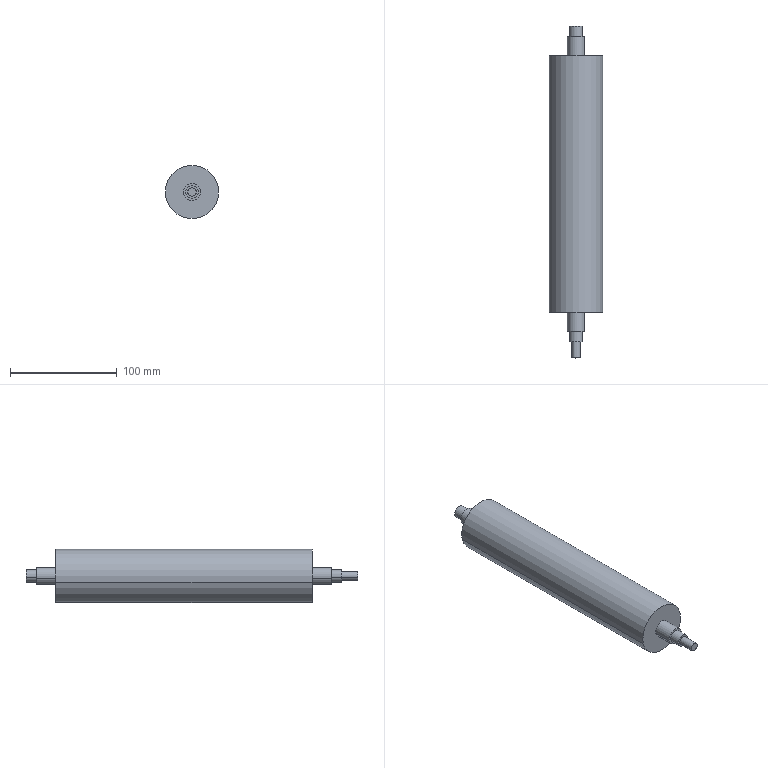Component | SolidWorks | AdjustmentRing-2 | 2 solids | 19 faces | box 50 x 311 x 50 mm | volume 481493 mm3 | cylinder 12 | plane 7 | commonest cylinder face diameters 16 x4 12 x4 50 x2 8 x2
build123d program:
from build123d import *

# Parameters (mm, degrees)
SKETCH4_R           = 25
SKETCH4_R_2         = 8
BOSS_EXTRUDE3_DEPTH = 120


with BuildPart() as part:
    # Sketch1 → Revolve1 (revolve)
    with BuildSketch(Plane.XY, mode=Mode.PRIVATE) as revolve1_sk:
        Polygon((0, 0), (6, 0), (6, 10), (8, 10), (8, 286), (6, 286), (6, 296), (4, 296), (4, 311), (0, 311), align=None)
    revolve(revolve1_sk.sketch.rotate(Axis((0, 0, 0), (0, 1, 0)), 90), axis=Axis((0, 0, 0), (0, 1, 0)))


with BuildPart() as body_2:
    # Sketch4 → Boss-Extrude3 (new, symmetric)
    with BuildSketch(Plane(origin=(0, 148, 0), x_dir=(-1, 0, 0), z_dir=(0, -1, 0))):
        with Locations(Location((0, 0, 0), (0, 0, 90))):
            Circle(SKETCH4_R)
        with Locations(Location((0, 0, 0), (0, 0, 90))):
            Circle(SKETCH4_R_2, mode=Mode.SUBTRACT)
    extrude(amount=BOSS_EXTRUDE3_DEPTH, both=True)


solid = Compound([part.part, body_2.part])

# Placed as in the assembly
solid = solid.moved(Location((-35, 148, 0), (180, 0, 0)))
STEP:
#1=COLOUR_RGB('',0.7922,0.8196,0.9333);
#2=FILL_AREA_STYLE_COLOUR('',#1);
#3=FILL_AREA_STYLE('',(#2));
#4=SURFACE_STYLE_FILL_AREA(#3);
#5=SURFACE_SIDE_STYLE('',(#4));
#6=SURFACE_STYLE_USAGE(.BOTH.,#5);
#7=PRESENTATION_STYLE_ASSIGNMENT((#6));
#8=CARTESIAN_POINT('',(-1.531,-6.417,-0.0381));
#9=VERTEX_POINT('',#8);
#10=CARTESIAN_POINT('',(-1.225,-6.417,0.0381));
#11=VERTEX_POINT('',#10);
#12=CARTESIAN_POINT('',(-1.378,-6.417,0.));
#13=DIRECTION('',(0.,1.,-0.));
#14=DIRECTION('',(-0.9703,0.,-0.2419));
#15=AXIS2_PLACEMENT_3D('',#12,#13,#14);
#16=CIRCLE('',#15,0.1575);
#17=EDGE_CURVE('',#9,#11,#16,.T.);
#18=ORIENTED_EDGE('',*,*,#17,.T.);
#19=CARTESIAN_POINT('',(-1.225,-5.827,0.0381));
#20=VERTEX_POINT('',#19);
#21=CARTESIAN_POINT('',(-1.225,5.827,0.0381));
#22=DIRECTION('',(0.,1.,-0.));
#23=VECTOR('',#22,39.37);
#24=LINE('',#21,#23);
#25=EDGE_CURVE('',#11,#20,#24,.T.);
#26=ORIENTED_EDGE('',*,*,#25,.T.);
#27=CARTESIAN_POINT('',(-1.531,-5.827,-0.0381));
#28=VERTEX_POINT('',#27);
#29=CARTESIAN_POINT('',(-1.378,-5.827,0.));
#30=DIRECTION('',(0.,1.,-0.));
#31=DIRECTION('',(-0.9703,0.,-0.2419));
#32=AXIS2_PLACEMENT_3D('',#29,#30,#31);
#33=CIRCLE('',#32,0.1575);
#34=EDGE_CURVE('',#28,#20,#33,.T.);
#35=ORIENTED_EDGE('',*,*,#34,.F.);
#36=CARTESIAN_POINT('',(-1.531,5.827,-0.0381));
#37=DIRECTION('',(0.,1.,-0.));
#38=VECTOR('',#37,39.37);
#39=LINE('',#36,#38);
#40=EDGE_CURVE('',#9,#28,#39,.T.);
#41=ORIENTED_EDGE('',*,*,#40,.F.);
#42=EDGE_LOOP('',(#18,#26,#35,#41));
#43=FACE_OUTER_BOUND('',#42,.T.);
#44=CARTESIAN_POINT('',(-1.378,5.827,0.));
#45=DIRECTION('',(0.,1.,-0.));
#46=DIRECTION('',(-0.9703,0.,-0.2419));
#47=AXIS2_PLACEMENT_3D('',#44,#45,#46);
#48=CYLINDRICAL_SURFACE('',#47,0.1575);
#49=ADVANCED_FACE('',(#43),#48,.T.);
#50=CARTESIAN_POINT('',(-1.607,-5.827,-0.05715));
#51=VERTEX_POINT('',#50);
#52=CARTESIAN_POINT('',(-1.149,-5.827,0.05715));
#53=VERTEX_POINT('',#52);
#54=CARTESIAN_POINT('',(-1.378,-5.827,0.));
#55=DIRECTION('',(0.,1.,-0.));
#56=DIRECTION('',(-0.9703,0.,-0.2419));
#57=AXIS2_PLACEMENT_3D('',#54,#55,#56);
#58=CIRCLE('',#57,0.2362);
#59=EDGE_CURVE('',#51,#53,#58,.T.);
#60=ORIENTED_EDGE('',*,*,#59,.T.);
#61=CARTESIAN_POINT('',(-1.149,-5.433,0.05715));
#62=VERTEX_POINT('',#61);
#63=CARTESIAN_POINT('',(-1.149,5.827,0.05715));
#64=DIRECTION('',(0.,1.,-0.));
#65=VECTOR('',#64,39.37);
#66=LINE('',#63,#65);
#67=EDGE_CURVE('',#53,#62,#66,.T.);
#68=ORIENTED_EDGE('',*,*,#67,.T.);
#69=CARTESIAN_POINT('',(-1.607,-5.433,-0.05715));
#70=VERTEX_POINT('',#69);
#71=CARTESIAN_POINT('',(-1.378,-5.433,0.));
#72=DIRECTION('',(0.,1.,-0.));
#73=DIRECTION('',(-0.9703,0.,-0.2419));
#74=AXIS2_PLACEMENT_3D('',#71,#72,#73);
#75=CIRCLE('',#74,0.2362);
#76=EDGE_CURVE('',#70,#62,#75,.T.);
#77=ORIENTED_EDGE('',*,*,#76,.F.);
#78=CARTESIAN_POINT('',(-1.607,5.827,-0.05715));
#79=DIRECTION('',(0.,1.,-0.));
#80=VECTOR('',#79,39.37);
#81=LINE('',#78,#80);
#82=EDGE_CURVE('',#51,#70,#81,.T.);
#83=ORIENTED_EDGE('',*,*,#82,.F.);
#84=EDGE_LOOP('',(#60,#68,#77,#83));
#85=FACE_OUTER_BOUND('',#84,.T.);
#86=CARTESIAN_POINT('',(-1.378,5.827,0.));
#87=DIRECTION('',(0.,1.,-0.));
#88=DIRECTION('',(-0.9703,0.,-0.2419));
#89=AXIS2_PLACEMENT_3D('',#86,#87,#88);
#90=CYLINDRICAL_SURFACE('',#89,0.2362);
#91=ADVANCED_FACE('',(#85),#90,.T.);
#92=CARTESIAN_POINT('',(-1.684,-5.433,-0.0762));
#93=VERTEX_POINT('',#92);
#94=CARTESIAN_POINT('',(-1.072,-5.433,0.0762));
#95=VERTEX_POINT('',#94);
#96=CARTESIAN_POINT('',(-1.378,-5.433,0.));
#97=DIRECTION('',(0.,1.,-0.));
#98=DIRECTION('',(-0.9703,0.,-0.2419));
#99=AXIS2_PLACEMENT_3D('',#96,#97,#98);
#100=CIRCLE('',#99,0.315);
#101=EDGE_CURVE('',#93,#95,#100,.T.);
#102=ORIENTED_EDGE('',*,*,#101,.T.);
#103=CARTESIAN_POINT('',(-1.072,5.433,0.0762));
#104=VERTEX_POINT('',#103);
#105=CARTESIAN_POINT('',(-1.072,5.827,0.0762));
#106=DIRECTION('',(0.,1.,-0.));
#107=VECTOR('',#106,39.37);
#108=LINE('',#105,#107);
#109=EDGE_CURVE('',#95,#104,#108,.T.);
#110=ORIENTED_EDGE('',*,*,#109,.T.);
#111=CARTESIAN_POINT('',(-1.684,5.433,-0.0762));
#112=VERTEX_POINT('',#111);
#113=CARTESIAN_POINT('',(-1.378,5.433,0.));
#114=DIRECTION('',(0.,1.,-0.));
#115=DIRECTION('',(-0.9703,0.,-0.2419));
#116=AXIS2_PLACEMENT_3D('',#113,#114,#115);
#117=CIRCLE('',#116,0.315);
#118=EDGE_CURVE('',#112,#104,#117,.T.);
#119=ORIENTED_EDGE('',*,*,#118,.F.);
#120=CARTESIAN_POINT('',(-1.684,5.827,-0.0762));
#121=DIRECTION('',(0.,1.,-0.));
#122=VECTOR('',#121,39.37);
#123=LINE('',#120,#122);
#124=EDGE_CURVE('',#93,#112,#123,.T.);
#125=ORIENTED_EDGE('',*,*,#124,.F.);
#126=EDGE_LOOP('',(#102,#110,#119,#125));
#127=FACE_OUTER_BOUND('',#126,.T.);
#128=CARTESIAN_POINT('',(-1.378,5.827,0.));
#129=DIRECTION('',(0.,1.,-0.));
#130=DIRECTION('',(-0.9703,0.,-0.2419));
#131=AXIS2_PLACEMENT_3D('',#128,#129,#130);
#132=CYLINDRICAL_SURFACE('',#131,0.315);
#133=ADVANCED_FACE('',(#127),#132,.T.);
#134=CARTESIAN_POINT('',(-1.607,5.433,-0.05715));
#135=VERTEX_POINT('',#134);
#136=CARTESIAN_POINT('',(-1.149,5.433,0.05715));
#137=VERTEX_POINT('',#136);
#138=CARTESIAN_POINT('',(-1.378,5.433,0.));
#139=DIRECTION('',(0.,1.,-0.));
#140=DIRECTION('',(-0.9703,0.,-0.2419));
#141=AXIS2_PLACEMENT_3D('',#138,#139,#140);
#142=CIRCLE('',#141,0.2362);
#143=EDGE_CURVE('',#135,#137,#142,.T.);
#144=ORIENTED_EDGE('',*,*,#143,.T.);
#145=CARTESIAN_POINT('',(-1.149,5.827,0.05715));
#146=VERTEX_POINT('',#145);
#147=CARTESIAN_POINT('',(-1.149,5.827,0.05715));
#148=DIRECTION('',(0.,1.,-0.));
#149=VECTOR('',#148,39.37);
#150=LINE('',#147,#149);
#151=EDGE_CURVE('',#137,#146,#150,.T.);
#152=ORIENTED_EDGE('',*,*,#151,.T.);
#153=CARTESIAN_POINT('',(-1.607,5.827,-0.05715));
#154=VERTEX_POINT('',#153);
#155=CARTESIAN_POINT('',(-1.378,5.827,0.));
#156=DIRECTION('',(0.,1.,-0.));
#157=DIRECTION('',(-0.9703,0.,-0.2419));
#158=AXIS2_PLACEMENT_3D('',#155,#156,#157);
#159=CIRCLE('',#158,0.2362);
#160=EDGE_CURVE('',#154,#146,#159,.T.);
#161=ORIENTED_EDGE('',*,*,#160,.F.);
#162=CARTESIAN_POINT('',(-1.607,5.827,-0.05715));
#163=DIRECTION('',(0.,1.,-0.));
#164=VECTOR('',#163,39.37);
#165=LINE('',#162,#164);
#166=EDGE_CURVE('',#135,#154,#165,.T.);
#167=ORIENTED_EDGE('',*,*,#166,.F.);
#168=EDGE_LOOP('',(#144,#152,#161,#167));
#169=FACE_OUTER_BOUND('',#168,.T.);
#170=CARTESIAN_POINT('',(-1.378,5.827,0.));
#171=DIRECTION('',(0.,1.,-0.));
#172=DIRECTION('',(-0.9703,0.,-0.2419));
#173=AXIS2_PLACEMENT_3D('',#170,#171,#172);
#174=CYLINDRICAL_SURFACE('',#173,0.2362);
#175=ADVANCED_FACE('',(#169),#174,.T.);
#176=ORIENTED_EDGE('',*,*,#160,.T.);
#177=CARTESIAN_POINT('',(-1.378,5.827,0.));
#178=DIRECTION('',(0.,1.,-0.));
#179=DIRECTION('',(-0.9703,0.,-0.2419));
#180=AXIS2_PLACEMENT_3D('',#177,#178,#179);
#181=CIRCLE('',#180,0.2362);
#182=EDGE_CURVE('',#146,#154,#181,.T.);
#183=ORIENTED_EDGE('',*,*,#182,.T.);
#184=EDGE_LOOP('',(#176,#183));
#185=FACE_OUTER_BOUND('',#184,.T.);
#186=CARTESIAN_POINT('',(-1.378,5.827,0.));
#187=DIRECTION('',(0.,1.,-0.));
#188=DIRECTION('',(-0.9703,-0.,-0.2419));
#189=AXIS2_PLACEMENT_3D('',#186,#187,#188);
#190=PLANE('',#189);
#191=ADVANCED_FACE('',(#185),#190,.T.);
#192=ORIENTED_EDGE('',*,*,#151,.F.);
#193=CARTESIAN_POINT('',(-1.378,5.433,0.));
#194=DIRECTION('',(0.,1.,-0.));
#195=DIRECTION('',(-0.9703,0.,-0.2419));
#196=AXIS2_PLACEMENT_3D('',#193,#194,#195);
#197=CIRCLE('',#196,0.2362);
#198=EDGE_CURVE('',#137,#135,#197,.T.);
#199=ORIENTED_EDGE('',*,*,#198,.T.);
#200=ORIENTED_EDGE('',*,*,#166,.T.);
#201=ORIENTED_EDGE('',*,*,#182,.F.);
#202=EDGE_LOOP('',(#192,#199,#200,#201));
#203=FACE_OUTER_BOUND('',#202,.T.);
#204=CARTESIAN_POINT('',(-1.378,5.827,0.));
#205=DIRECTION('',(0.,1.,-0.));
#206=DIRECTION('',(-0.9703,0.,-0.2419));
#207=AXIS2_PLACEMENT_3D('',#204,#205,#206);
#208=CYLINDRICAL_SURFACE('',#207,0.2362);
#209=ADVANCED_FACE('',(#203),#208,.T.);
#210=ORIENTED_EDGE('',*,*,#118,.T.);
#211=CARTESIAN_POINT('',(-1.378,5.433,0.));
#212=DIRECTION('',(0.,1.,-0.));
#213=DIRECTION('',(-0.9703,0.,-0.2419));
#214=AXIS2_PLACEMENT_3D('',#211,#212,#213);
#215=CIRCLE('',#214,0.315);
#216=EDGE_CURVE('',#104,#112,#215,.T.);
#217=ORIENTED_EDGE('',*,*,#216,.T.);
#218=EDGE_LOOP('',(#210,#217));
#219=FACE_OUTER_BOUND('',#218,.T.);
#220=ORIENTED_EDGE('',*,*,#143,.F.);
#221=ORIENTED_EDGE('',*,*,#198,.F.);
#222=EDGE_LOOP('',(#220,#221));
#223=FACE_BOUND('',#222,.T.);
#224=CARTESIAN_POINT('',(-1.435,5.433,0.2292));
#225=DIRECTION('',(0.,1.,-0.));
#226=DIRECTION('',(-0.9703,-0.,-0.2419));
#227=AXIS2_PLACEMENT_3D('',#224,#225,#226);
#228=PLANE('',#227);
#229=ADVANCED_FACE('',(#219,#223),#228,.T.);
#230=ORIENTED_EDGE('',*,*,#109,.F.);
#231=CARTESIAN_POINT('',(-1.378,-5.433,0.));
#232=DIRECTION('',(0.,1.,-0.));
#233=DIRECTION('',(-0.9703,0.,-0.2419));
#234=AXIS2_PLACEMENT_3D('',#231,#232,#233);
#235=CIRCLE('',#234,0.315);
#236=EDGE_CURVE('',#95,#93,#235,.T.);
#237=ORIENTED_EDGE('',*,*,#236,.T.);
#238=ORIENTED_EDGE('',*,*,#124,.T.);
#239=ORIENTED_EDGE('',*,*,#216,.F.);
#240=EDGE_LOOP('',(#230,#237,#238,#239));
#241=FACE_OUTER_BOUND('',#240,.T.);
#242=CARTESIAN_POINT('',(-1.378,5.827,0.));
#243=DIRECTION('',(0.,1.,-0.));
#244=DIRECTION('',(-0.9703,0.,-0.2419));
#245=AXIS2_PLACEMENT_3D('',#242,#243,#244);
#246=CYLINDRICAL_SURFACE('',#245,0.315);
#247=ADVANCED_FACE('',(#241),#246,.T.);
#248=ORIENTED_EDGE('',*,*,#76,.T.);
#249=CARTESIAN_POINT('',(-1.378,-5.433,0.));
#250=DIRECTION('',(0.,1.,-0.));
#251=DIRECTION('',(-0.9703,0.,-0.2419));
#252=AXIS2_PLACEMENT_3D('',#249,#250,#251);
#253=CIRCLE('',#252,0.2362);
#254=EDGE_CURVE('',#62,#70,#253,.T.);
#255=ORIENTED_EDGE('',*,*,#254,.T.);
#256=EDGE_LOOP('',(#248,#255));
#257=FACE_BOUND('',#256,.T.);
#258=ORIENTED_EDGE('',*,*,#101,.F.);
#259=ORIENTED_EDGE('',*,*,#236,.F.);
#260=EDGE_LOOP('',(#258,#259));
#261=FACE_OUTER_BOUND('',#260,.T.);
#262=CARTESIAN_POINT('',(-1.454,-5.433,0.3056));
#263=DIRECTION('',(-0.,-1.,0.));
#264=DIRECTION('',(0.9703,0.,0.2419));
#265=AXIS2_PLACEMENT_3D('',#262,#263,#264);
#266=PLANE('',#265);
#267=ADVANCED_FACE('',(#257,#261),#266,.T.);
#268=ORIENTED_EDGE('',*,*,#67,.F.);
#269=CARTESIAN_POINT('',(-1.378,-5.827,0.));
#270=DIRECTION('',(0.,1.,-0.));
#271=DIRECTION('',(-0.9703,0.,-0.2419));
#272=AXIS2_PLACEMENT_3D('',#269,#270,#271);
#273=CIRCLE('',#272,0.2362);
#274=EDGE_CURVE('',#53,#51,#273,.T.);
#275=ORIENTED_EDGE('',*,*,#274,.T.);
#276=ORIENTED_EDGE('',*,*,#82,.T.);
#277=ORIENTED_EDGE('',*,*,#254,.F.);
#278=EDGE_LOOP('',(#268,#275,#276,#277));
#279=FACE_OUTER_BOUND('',#278,.T.);
#280=CARTESIAN_POINT('',(-1.378,5.827,0.));
#281=DIRECTION('',(0.,1.,-0.));
#282=DIRECTION('',(-0.9703,0.,-0.2419));
#283=AXIS2_PLACEMENT_3D('',#280,#281,#282);
#284=CYLINDRICAL_SURFACE('',#283,0.2362);
#285=ADVANCED_FACE('',(#279),#284,.T.);
#286=ORIENTED_EDGE('',*,*,#34,.T.);
#287=CARTESIAN_POINT('',(-1.378,-5.827,0.));
#288=DIRECTION('',(0.,1.,-0.));
#289=DIRECTION('',(-0.9703,0.,-0.2419));
#290=AXIS2_PLACEMENT_3D('',#287,#288,#289);
#291=CIRCLE('',#290,0.1575);
#292=EDGE_CURVE('',#20,#28,#291,.T.);
#293=ORIENTED_EDGE('',*,*,#292,.T.);
#294=EDGE_LOOP('',(#286,#293));
#295=FACE_BOUND('',#294,.T.);
#296=ORIENTED_EDGE('',*,*,#59,.F.);
#297=ORIENTED_EDGE('',*,*,#274,.F.);
#298=EDGE_LOOP('',(#296,#297));
#299=FACE_OUTER_BOUND('',#298,.T.);
#300=CARTESIAN_POINT('',(-1.435,-5.827,0.2292));
#301=DIRECTION('',(-0.,-1.,0.));
#302=DIRECTION('',(0.9703,0.,0.2419));
#303=AXIS2_PLACEMENT_3D('',#300,#301,#302);
#304=PLANE('',#303);
#305=ADVANCED_FACE('',(#295,#299),#304,.T.);
#306=ORIENTED_EDGE('',*,*,#25,.F.);
#307=CARTESIAN_POINT('',(-1.378,-6.417,0.));
#308=DIRECTION('',(0.,1.,-0.));
#309=DIRECTION('',(-0.9703,0.,-0.2419));
#310=AXIS2_PLACEMENT_3D('',#307,#308,#309);
#311=CIRCLE('',#310,0.1575);
#312=EDGE_CURVE('',#11,#9,#311,.T.);
#313=ORIENTED_EDGE('',*,*,#312,.T.);
#314=ORIENTED_EDGE('',*,*,#40,.T.);
#315=ORIENTED_EDGE('',*,*,#292,.F.);
#316=EDGE_LOOP('',(#306,#313,#314,#315));
#317=FACE_OUTER_BOUND('',#316,.T.);
#318=CARTESIAN_POINT('',(-1.378,5.827,0.));
#319=DIRECTION('',(0.,1.,-0.));
#320=DIRECTION('',(-0.9703,0.,-0.2419));
#321=AXIS2_PLACEMENT_3D('',#318,#319,#320);
#322=CYLINDRICAL_SURFACE('',#321,0.1575);
#323=ADVANCED_FACE('',(#317),#322,.T.);
#324=ORIENTED_EDGE('',*,*,#17,.F.);
#325=ORIENTED_EDGE('',*,*,#312,.F.);
#326=EDGE_LOOP('',(#324,#325));
#327=FACE_OUTER_BOUND('',#326,.T.);
#328=CARTESIAN_POINT('',(-1.416,-6.417,0.1528));
#329=DIRECTION('',(-0.,-1.,0.));
#330=DIRECTION('',(0.9703,0.,0.2419));
#331=AXIS2_PLACEMENT_3D('',#328,#329,#330);
#332=PLANE('',#331);
#333=ADVANCED_FACE('',(#327),#332,.T.);
#334=CLOSED_SHELL('',(#49,#91,#133,#175,#191,#209,#229,#247,#267,#285,#305,#323,#333));
#335=MANIFOLD_SOLID_BREP('',#334);
#336=STYLED_ITEM('',(#7),#335);
#337=PRESENTATION_LAYER_ASSIGNMENT('','',(#336));
#338=CARTESIAN_POINT('',(-1.072,4.724,0.0762));
#339=VERTEX_POINT('',#338);
#340=CARTESIAN_POINT('',(-1.684,4.724,-0.0762));
#341=VERTEX_POINT('',#340);
#342=CARTESIAN_POINT('',(-1.378,4.724,0.));
#343=DIRECTION('',(0.,1.,-0.));
#344=DIRECTION('',(-0.9703,0.,-0.2419));
#345=AXIS2_PLACEMENT_3D('',#342,#343,#344);
#346=CIRCLE('',#345,0.315);
#347=EDGE_CURVE('',#339,#341,#346,.T.);
#348=ORIENTED_EDGE('',*,*,#347,.T.);
#349=CARTESIAN_POINT('',(-1.684,-4.724,-0.0762));
#350=VERTEX_POINT('',#349);
#351=CARTESIAN_POINT('',(-1.684,4.724,-0.0762));
#352=DIRECTION('',(-0.,-1.,0.));
#353=VECTOR('',#352,39.37);
#354=LINE('',#351,#353);
#355=EDGE_CURVE('',#341,#350,#354,.T.);
#356=ORIENTED_EDGE('',*,*,#355,.T.);
#357=CARTESIAN_POINT('',(-1.072,-4.724,0.0762));
#358=VERTEX_POINT('',#357);
#359=CARTESIAN_POINT('',(-1.378,-4.724,0.));
#360=DIRECTION('',(0.,1.,-0.));
#361=DIRECTION('',(-0.9703,0.,-0.2419));
#362=AXIS2_PLACEMENT_3D('',#359,#360,#361);
#363=CIRCLE('',#362,0.315);
#364=EDGE_CURVE('',#358,#350,#363,.T.);
#365=ORIENTED_EDGE('',*,*,#364,.F.);
#366=CARTESIAN_POINT('',(-1.072,4.724,0.0762));
#367=DIRECTION('',(-0.,-1.,0.));
#368=VECTOR('',#367,39.37);
#369=LINE('',#366,#368);
#370=EDGE_CURVE('',#339,#358,#369,.T.);
#371=ORIENTED_EDGE('',*,*,#370,.F.);
#372=EDGE_LOOP('',(#348,#356,#365,#371));
#373=FACE_OUTER_BOUND('',#372,.T.);
#374=CARTESIAN_POINT('',(-1.378,4.724,0.));
#375=DIRECTION('',(-0.,-1.,0.));
#376=DIRECTION('',(0.9703,0.,0.2419));
#377=AXIS2_PLACEMENT_3D('',#374,#375,#376);
#378=CYLINDRICAL_SURFACE('',#377,0.315);
#379=ADVANCED_FACE('',(#373),#378,.F.);
#380=CARTESIAN_POINT('',(-2.333,4.724,-0.2381));
#381=VERTEX_POINT('',#380);
#382=CARTESIAN_POINT('',(-0.4229,4.724,0.2381));
#383=VERTEX_POINT('',#382);
#384=CARTESIAN_POINT('',(-1.378,4.724,0.));
#385=DIRECTION('',(0.,1.,-0.));
#386=DIRECTION('',(-0.9703,0.,-0.2419));
#387=AXIS2_PLACEMENT_3D('',#384,#385,#386);
#388=CIRCLE('',#387,0.9843);
#389=EDGE_CURVE('',#381,#383,#388,.T.);
#390=ORIENTED_EDGE('',*,*,#389,.F.);
#391=CARTESIAN_POINT('',(-2.333,-4.724,-0.2381));
#392=VERTEX_POINT('',#391);
#393=CARTESIAN_POINT('',(-2.333,4.724,-0.2381));
#394=DIRECTION('',(-0.,-1.,0.));
#395=VECTOR('',#394,39.37);
#396=LINE('',#393,#395);
#397=EDGE_CURVE('',#381,#392,#396,.T.);
#398=ORIENTED_EDGE('',*,*,#397,.T.);
#399=CARTESIAN_POINT('',(-0.4229,-4.724,0.2381));
#400=VERTEX_POINT('',#399);
#401=CARTESIAN_POINT('',(-1.378,-4.724,0.));
#402=DIRECTION('',(0.,1.,-0.));
#403=DIRECTION('',(-0.9703,0.,-0.2419));
#404=AXIS2_PLACEMENT_3D('',#401,#402,#403);
#405=CIRCLE('',#404,0.9843);
#406=EDGE_CURVE('',#392,#400,#405,.T.);
#407=ORIENTED_EDGE('',*,*,#406,.T.);
#408=CARTESIAN_POINT('',(-0.4229,4.724,0.2381));
#409=DIRECTION('',(-0.,-1.,0.));
#410=VECTOR('',#409,39.37);
#411=LINE('',#408,#410);
#412=EDGE_CURVE('',#383,#400,#411,.T.);
#413=ORIENTED_EDGE('',*,*,#412,.F.);
#414=EDGE_LOOP('',(#390,#398,#407,#413));
#415=FACE_OUTER_BOUND('',#414,.T.);
#416=CARTESIAN_POINT('',(-1.378,4.724,0.));
#417=DIRECTION('',(-0.,-1.,0.));
#418=DIRECTION('',(0.9703,0.,0.2419));
#419=AXIS2_PLACEMENT_3D('',#416,#417,#418);
#420=CYLINDRICAL_SURFACE('',#419,0.9843);
#421=ADVANCED_FACE('',(#415),#420,.T.);
#422=CARTESIAN_POINT('',(-1.378,4.724,0.));
#423=DIRECTION('',(0.,1.,-0.));
#424=DIRECTION('',(-0.9703,0.,-0.2419));
#425=AXIS2_PLACEMENT_3D('',#422,#423,#424);
#426=CIRCLE('',#425,0.9843);
#427=EDGE_CURVE('',#383,#381,#426,.T.);
#428=ORIENTED_EDGE('',*,*,#427,.T.);
#429=ORIENTED_EDGE('',*,*,#389,.T.);
#430=EDGE_LOOP('',(#428,#429));
#431=FACE_OUTER_BOUND('',#430,.T.);
#432=ORIENTED_EDGE('',*,*,#347,.F.);
#433=CARTESIAN_POINT('',(-1.378,4.724,0.));
#434=DIRECTION('',(0.,1.,-0.));
#435=DIRECTION('',(-0.9703,0.,-0.2419));
#436=AXIS2_PLACEMENT_3D('',#433,#434,#435);
#437=CIRCLE('',#436,0.315);
#438=EDGE_CURVE('',#341,#339,#437,.T.);
#439=ORIENTED_EDGE('',*,*,#438,.F.);
#440=EDGE_LOOP('',(#432,#439));
#441=FACE_BOUND('',#440,.T.);
#442=CARTESIAN_POINT('',(-1.378,4.724,0.));
#443=DIRECTION('',(0.,1.,-0.));
#444=DIRECTION('',(-0.9703,-0.,-0.2419));
#445=AXIS2_PLACEMENT_3D('',#442,#443,#444);
#446=PLANE('',#445);
#447=ADVANCED_FACE('',(#431,#441),#446,.T.);
#448=CARTESIAN_POINT('',(-1.378,-4.724,0.));
#449=DIRECTION('',(0.,1.,-0.));
#450=DIRECTION('',(-0.9703,0.,-0.2419));
#451=AXIS2_PLACEMENT_3D('',#448,#449,#450);
#452=CIRCLE('',#451,0.9843);
#453=EDGE_CURVE('',#400,#392,#452,.T.);
#454=ORIENTED_EDGE('',*,*,#453,.F.);
#455=ORIENTED_EDGE('',*,*,#406,.F.);
#456=EDGE_LOOP('',(#454,#455));
#457=FACE_OUTER_BOUND('',#456,.T.);
#458=ORIENTED_EDGE('',*,*,#364,.T.);
#459=CARTESIAN_POINT('',(-1.378,-4.724,0.));
#460=DIRECTION('',(0.,1.,-0.));
#461=DIRECTION('',(-0.9703,0.,-0.2419));
#462=AXIS2_PLACEMENT_3D('',#459,#460,#461);
#463=CIRCLE('',#462,0.315);
#464=EDGE_CURVE('',#350,#358,#463,.T.);
#465=ORIENTED_EDGE('',*,*,#464,.T.);
#466=EDGE_LOOP('',(#458,#465));
#467=FACE_BOUND('',#466,.T.);
#468=CARTESIAN_POINT('',(-1.378,-4.724,0.));
#469=DIRECTION('',(0.,1.,-0.));
#470=DIRECTION('',(-0.9703,-0.,-0.2419));
#471=AXIS2_PLACEMENT_3D('',#468,#469,#470);
#472=PLANE('',#471);
#473=ADVANCED_FACE('',(#457,#467),#472,.F.);
#474=ORIENTED_EDGE('',*,*,#397,.F.);
#475=ORIENTED_EDGE('',*,*,#427,.F.);
#476=ORIENTED_EDGE('',*,*,#412,.T.);
#477=ORIENTED_EDGE('',*,*,#453,.T.);
#478=EDGE_LOOP('',(#474,#475,#476,#477));
#479=FACE_OUTER_BOUND('',#478,.T.);
#480=CARTESIAN_POINT('',(-1.378,4.724,0.));
#481=DIRECTION('',(-0.,-1.,0.));
#482=DIRECTION('',(0.9703,0.,0.2419));
#483=AXIS2_PLACEMENT_3D('',#480,#481,#482);
#484=CYLINDRICAL_SURFACE('',#483,0.9843);
#485=ADVANCED_FACE('',(#479),#484,.T.);
#486=ORIENTED_EDGE('',*,*,#355,.F.);
#487=ORIENTED_EDGE('',*,*,#438,.T.);
#488=ORIENTED_EDGE('',*,*,#370,.T.);
#489=ORIENTED_EDGE('',*,*,#464,.F.);
#490=EDGE_LOOP('',(#486,#487,#488,#489));
#491=FACE_OUTER_BOUND('',#490,.T.);
#492=CARTESIAN_POINT('',(-1.378,4.724,0.));
#493=DIRECTION('',(-0.,-1.,0.));
#494=DIRECTION('',(0.9703,0.,0.2419));
#495=AXIS2_PLACEMENT_3D('',#492,#493,#494);
#496=CYLINDRICAL_SURFACE('',#495,0.315);
#497=ADVANCED_FACE('',(#491),#496,.F.);
#498=CLOSED_SHELL('',(#379,#421,#447,#473,#485,#497));
#499=MANIFOLD_SOLID_BREP('',#498);
#500=CARTESIAN_POINT('',(0.,0.,0.));
#501=DIRECTION('',(0.,0.,1.));
#502=DIRECTION('',(1.,0.,0.));
#503=AXIS2_PLACEMENT_3D('',#500,#501,#502);
#504=(LENGTH_UNIT()NAMED_UNIT(*)SI_UNIT($,.METRE.));
#505=LENGTH_MEASURE_WITH_UNIT(LENGTH_MEASURE(0.0254),#504);
#506=DIMENSIONAL_EXPONENTS(1.,0.,0.,0.,0.,0.,0.);
#507=(CONVERSION_BASED_UNIT('',#505)LENGTH_UNIT()NAMED_UNIT(#506));
#508=UNCERTAINTY_MEASURE_WITH_UNIT(LENGTH_MEASURE(0.00001),#507,'','');
#509=(NAMED_UNIT(*)PLANE_ANGLE_UNIT()SI_UNIT($,.RADIAN.));
#510=(NAMED_UNIT(*)SI_UNIT($,.STERADIAN.)SOLID_ANGLE_UNIT());
#511=(GEOMETRIC_REPRESENTATION_CONTEXT(3)GLOBAL_UNCERTAINTY_ASSIGNED_CONTEXT((#508))GLOBAL_UNIT_ASSIGNED_CONTEXT((#507,#509,#510))REPRESENTATION_CONTEXT('',''));
#512=ADVANCED_BREP_SHAPE_REPRESENTATION('',(#499,#335,#503),#511);
#513=COLOUR_RGB('',0.7922,0.8196,0.9333);
#514=FILL_AREA_STYLE_COLOUR('',#513);
#515=FILL_AREA_STYLE('',(#514));
#516=SURFACE_STYLE_FILL_AREA(#515);
#517=SURFACE_SIDE_STYLE('',(#516));
#518=SURFACE_STYLE_USAGE(.BOTH.,#517);
#519=PRESENTATION_STYLE_ASSIGNMENT((#518));
#520=STYLED_ITEM('',(#519),#499);
#521=(LENGTH_UNIT()NAMED_UNIT(*)SI_UNIT($,.METRE.));
#522=LENGTH_MEASURE_WITH_UNIT(LENGTH_MEASURE(0.0254),#521);
#523=DIMENSIONAL_EXPONENTS(1.,0.,0.,0.,0.,0.,0.);
#524=(CONVERSION_BASED_UNIT('',#522)LENGTH_UNIT()NAMED_UNIT(#523));
#525=UNCERTAINTY_MEASURE_WITH_UNIT(LENGTH_MEASURE(0.00001),#524,'','');
#526=(NAMED_UNIT(*)PLANE_ANGLE_UNIT()SI_UNIT($,.RADIAN.));
#527=(NAMED_UNIT(*)SI_UNIT($,.STERADIAN.)SOLID_ANGLE_UNIT());
#528=(GEOMETRIC_REPRESENTATION_CONTEXT(3)GLOBAL_UNCERTAINTY_ASSIGNED_CONTEXT((#525))GLOBAL_UNIT_ASSIGNED_CONTEXT((#524,#526,#527))REPRESENTATION_CONTEXT('',''));
#529=MECHANICAL_DESIGN_GEOMETRIC_PRESENTATION_REPRESENTATION('',(#520),#528);
#530=PRESENTATION_LAYER_ASSIGNMENT('','',(#520));
#531=(LENGTH_UNIT()NAMED_UNIT(*)SI_UNIT($,.METRE.));
#532=LENGTH_MEASURE_WITH_UNIT(LENGTH_MEASURE(0.0254),#531);
#533=DIMENSIONAL_EXPONENTS(1.,0.,0.,0.,0.,0.,0.);
#534=(CONVERSION_BASED_UNIT('',#532)LENGTH_UNIT()NAMED_UNIT(#533));
#535=UNCERTAINTY_MEASURE_WITH_UNIT(LENGTH_MEASURE(0.00001),#534,'','');
#536=(NAMED_UNIT(*)PLANE_ANGLE_UNIT()SI_UNIT($,.RADIAN.));
#537=(NAMED_UNIT(*)SI_UNIT($,.STERADIAN.)SOLID_ANGLE_UNIT());
#538=(GEOMETRIC_REPRESENTATION_CONTEXT(3)GLOBAL_UNCERTAINTY_ASSIGNED_CONTEXT((#535))GLOBAL_UNIT_ASSIGNED_CONTEXT((#534,#536,#537))REPRESENTATION_CONTEXT('',''));
#539=MECHANICAL_DESIGN_GEOMETRIC_PRESENTATION_REPRESENTATION('',(#336),#538);